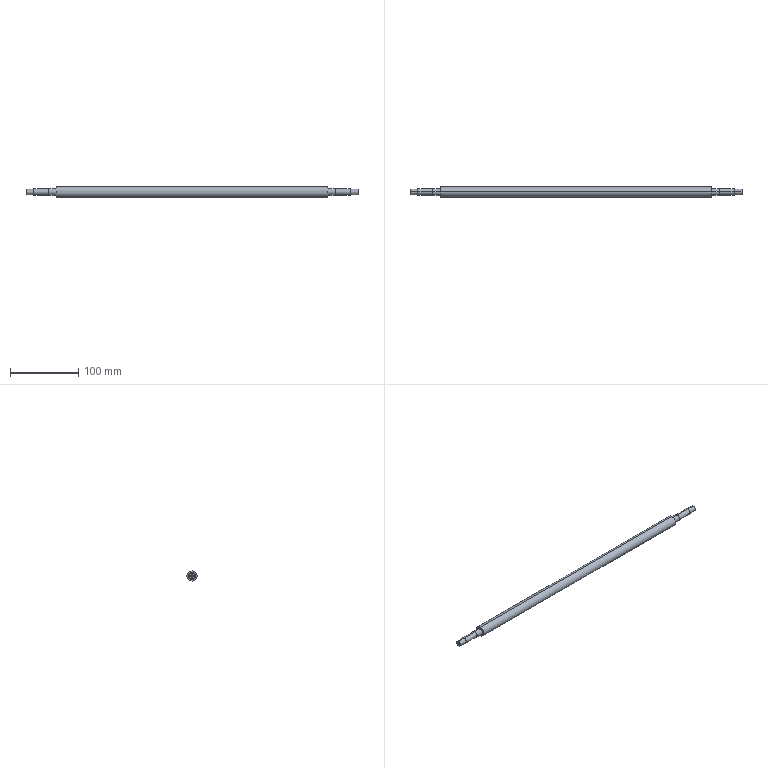Component | SolidWorks | PushRod3-1 | 1 solid | 28 faces | box 487 x 15 x 15 mm | volume 75810 mm3 | cylinder 18 | plane 10 | commonest cylinder face diameters 8 x4 3.3 x4 9 x4 10 x4 15 x2
STEP:
#1=COLOUR_RGB('',0.7922,0.8196,0.9333);
#2=FILL_AREA_STYLE_COLOUR('',#1);
#3=FILL_AREA_STYLE('',(#2));
#4=SURFACE_STYLE_FILL_AREA(#3);
#5=SURFACE_SIDE_STYLE('',(#4));
#6=SURFACE_STYLE_USAGE(.BOTH.,#5);
#7=PRESENTATION_STYLE_ASSIGNMENT((#6));
#8=CARTESIAN_POINT('',(9.587,5.032,2.961));
#9=VERTEX_POINT('',#8);
#10=CARTESIAN_POINT('',(9.587,5.032,3.276));
#11=VERTEX_POINT('',#10);
#12=CARTESIAN_POINT('',(9.587,5.032,3.119));
#13=DIRECTION('',(1.,0.,0.));
#14=DIRECTION('',(0.,0.,-1.));
#15=AXIS2_PLACEMENT_3D('',#12,#13,#14);
#16=CIRCLE('',#15,0.1575);
#17=EDGE_CURVE('',#9,#11,#16,.T.);
#18=ORIENTED_EDGE('',*,*,#17,.F.);
#19=CARTESIAN_POINT('',(9.134,5.032,2.961));
#20=VERTEX_POINT('',#19);
#21=CARTESIAN_POINT('',(9.587,5.032,2.961));
#22=DIRECTION('',(-1.,0.,0.));
#23=VECTOR('',#22,39.37);
#24=LINE('',#21,#23);
#25=EDGE_CURVE('',#9,#20,#24,.T.);
#26=ORIENTED_EDGE('',*,*,#25,.T.);
#27=CARTESIAN_POINT('',(9.134,5.032,3.276));
#28=VERTEX_POINT('',#27);
#29=CARTESIAN_POINT('',(9.134,5.032,3.119));
#30=DIRECTION('',(1.,0.,0.));
#31=DIRECTION('',(0.,0.,-1.));
#32=AXIS2_PLACEMENT_3D('',#29,#30,#31);
#33=CIRCLE('',#32,0.1575);
#34=EDGE_CURVE('',#20,#28,#33,.T.);
#35=ORIENTED_EDGE('',*,*,#34,.T.);
#36=CARTESIAN_POINT('',(9.587,5.032,3.276));
#37=DIRECTION('',(-1.,0.,0.));
#38=VECTOR('',#37,39.37);
#39=LINE('',#36,#38);
#40=EDGE_CURVE('',#11,#28,#39,.T.);
#41=ORIENTED_EDGE('',*,*,#40,.F.);
#42=EDGE_LOOP('',(#18,#26,#35,#41));
#43=FACE_OUTER_BOUND('',#42,.T.);
#44=CARTESIAN_POINT('',(9.587,5.032,3.119));
#45=DIRECTION('',(-1.,0.,0.));
#46=DIRECTION('',(0.,0.,1.));
#47=AXIS2_PLACEMENT_3D('',#44,#45,#46);
#48=CYLINDRICAL_SURFACE('',#47,0.1575);
#49=ADVANCED_FACE('',(#43),#48,.T.);
#50=CARTESIAN_POINT('',(9.114,5.032,3.184));
#51=VERTEX_POINT('',#50);
#52=CARTESIAN_POINT('',(9.114,5.032,3.054));
#53=VERTEX_POINT('',#52);
#54=CARTESIAN_POINT('',(9.114,5.032,3.119));
#55=DIRECTION('',(1.,0.,0.));
#56=DIRECTION('',(0.,0.,-1.));
#57=AXIS2_PLACEMENT_3D('',#54,#55,#56);
#58=CIRCLE('',#57,0.06496);
#59=EDGE_CURVE('',#51,#53,#58,.T.);
#60=ORIENTED_EDGE('',*,*,#59,.F.);
#61=CARTESIAN_POINT('',(9.587,5.032,3.184));
#62=VERTEX_POINT('',#61);
#63=CARTESIAN_POINT('',(9.114,5.032,3.184));
#64=DIRECTION('',(1.,0.,0.));
#65=VECTOR('',#64,39.37);
#66=LINE('',#63,#65);
#67=EDGE_CURVE('',#51,#62,#66,.T.);
#68=ORIENTED_EDGE('',*,*,#67,.T.);
#69=CARTESIAN_POINT('',(9.587,5.032,3.054));
#70=VERTEX_POINT('',#69);
#71=CARTESIAN_POINT('',(9.587,5.032,3.119));
#72=DIRECTION('',(1.,0.,0.));
#73=DIRECTION('',(0.,0.,-1.));
#74=AXIS2_PLACEMENT_3D('',#71,#72,#73);
#75=CIRCLE('',#74,0.06496);
#76=EDGE_CURVE('',#62,#70,#75,.T.);
#77=ORIENTED_EDGE('',*,*,#76,.T.);
#78=CARTESIAN_POINT('',(9.114,5.032,3.054));
#79=DIRECTION('',(1.,0.,0.));
#80=VECTOR('',#79,39.37);
#81=LINE('',#78,#80);
#82=EDGE_CURVE('',#53,#70,#81,.T.);
#83=ORIENTED_EDGE('',*,*,#82,.F.);
#84=EDGE_LOOP('',(#60,#68,#77,#83));
#85=FACE_OUTER_BOUND('',#84,.T.);
#86=CARTESIAN_POINT('',(9.114,5.032,3.119));
#87=DIRECTION('',(1.,0.,0.));
#88=DIRECTION('',(0.,0.,-1.));
#89=AXIS2_PLACEMENT_3D('',#86,#87,#88);
#90=CYLINDRICAL_SURFACE('',#89,0.06496);
#91=ADVANCED_FACE('',(#85),#90,.F.);
#92=CARTESIAN_POINT('',(8.268,5.032,3.296));
#93=VERTEX_POINT('',#92);
#94=CARTESIAN_POINT('',(8.268,5.032,2.941));
#95=VERTEX_POINT('',#94);
#96=CARTESIAN_POINT('',(8.268,5.032,3.119));
#97=DIRECTION('',(-1.,0.,0.));
#98=DIRECTION('',(0.,0.,1.));
#99=AXIS2_PLACEMENT_3D('',#96,#97,#98);
#100=CIRCLE('',#99,0.1772);
#101=EDGE_CURVE('',#93,#95,#100,.T.);
#102=ORIENTED_EDGE('',*,*,#101,.F.);
#103=CARTESIAN_POINT('',(9.134,5.032,3.296));
#104=VERTEX_POINT('',#103);
#105=CARTESIAN_POINT('',(8.228,5.032,3.296));
#106=DIRECTION('',(1.,0.,0.));
#107=VECTOR('',#106,39.37);
#108=LINE('',#105,#107);
#109=EDGE_CURVE('',#93,#104,#108,.T.);
#110=ORIENTED_EDGE('',*,*,#109,.T.);
#111=CARTESIAN_POINT('',(9.134,5.032,2.941));
#112=VERTEX_POINT('',#111);
#113=CARTESIAN_POINT('',(9.134,5.032,3.119));
#114=DIRECTION('',(1.,0.,0.));
#115=DIRECTION('',(0.,0.,-1.));
#116=AXIS2_PLACEMENT_3D('',#113,#114,#115);
#117=CIRCLE('',#116,0.1772);
#118=EDGE_CURVE('',#112,#104,#117,.T.);
#119=ORIENTED_EDGE('',*,*,#118,.F.);
#120=CARTESIAN_POINT('',(8.228,5.032,2.941));
#121=DIRECTION('',(1.,0.,0.));
#122=VECTOR('',#121,39.37);
#123=LINE('',#120,#122);
#124=EDGE_CURVE('',#95,#112,#123,.T.);
#125=ORIENTED_EDGE('',*,*,#124,.F.);
#126=EDGE_LOOP('',(#102,#110,#119,#125));
#127=FACE_OUTER_BOUND('',#126,.T.);
#128=CARTESIAN_POINT('',(8.228,5.032,3.119));
#129=DIRECTION('',(1.,0.,0.));
#130=DIRECTION('',(0.,0.,-1.));
#131=AXIS2_PLACEMENT_3D('',#128,#129,#130);
#132=CYLINDRICAL_SURFACE('',#131,0.1772);
#133=ADVANCED_FACE('',(#127),#132,.T.);
#134=CARTESIAN_POINT('',(8.268,5.032,3.315));
#135=VERTEX_POINT('',#134);
#136=CARTESIAN_POINT('',(8.268,5.032,2.922));
#137=VERTEX_POINT('',#136);
#138=CARTESIAN_POINT('',(8.268,5.032,3.119));
#139=DIRECTION('',(-1.,0.,0.));
#140=DIRECTION('',(0.,0.,1.));
#141=AXIS2_PLACEMENT_3D('',#138,#139,#140);
#142=CIRCLE('',#141,0.1969);
#143=EDGE_CURVE('',#135,#137,#142,.T.);
#144=ORIENTED_EDGE('',*,*,#143,.T.);
#145=CARTESIAN_POINT('',(7.835,5.032,2.922));
#146=VERTEX_POINT('',#145);
#147=CARTESIAN_POINT('',(9.134,5.032,2.922));
#148=DIRECTION('',(-1.,0.,0.));
#149=VECTOR('',#148,39.37);
#150=LINE('',#147,#149);
#151=EDGE_CURVE('',#137,#146,#150,.T.);
#152=ORIENTED_EDGE('',*,*,#151,.T.);
#153=CARTESIAN_POINT('',(7.835,5.032,3.315));
#154=VERTEX_POINT('',#153);
#155=CARTESIAN_POINT('',(7.835,5.032,3.119));
#156=DIRECTION('',(1.,0.,0.));
#157=DIRECTION('',(0.,0.,-1.));
#158=AXIS2_PLACEMENT_3D('',#155,#156,#157);
#159=CIRCLE('',#158,0.1969);
#160=EDGE_CURVE('',#146,#154,#159,.T.);
#161=ORIENTED_EDGE('',*,*,#160,.T.);
#162=CARTESIAN_POINT('',(9.134,5.032,3.315));
#163=DIRECTION('',(-1.,0.,0.));
#164=VECTOR('',#163,39.37);
#165=LINE('',#162,#164);
#166=EDGE_CURVE('',#135,#154,#165,.T.);
#167=ORIENTED_EDGE('',*,*,#166,.F.);
#168=EDGE_LOOP('',(#144,#152,#161,#167));
#169=FACE_OUTER_BOUND('',#168,.T.);
#170=CARTESIAN_POINT('',(9.134,5.032,3.119));
#171=DIRECTION('',(-1.,0.,0.));
#172=DIRECTION('',(0.,0.,1.));
#173=AXIS2_PLACEMENT_3D('',#170,#171,#172);
#174=CYLINDRICAL_SURFACE('',#173,0.1969);
#175=ADVANCED_FACE('',(#169),#174,.T.);
#176=CARTESIAN_POINT('',(7.835,5.032,2.823));
#177=VERTEX_POINT('',#176);
#178=CARTESIAN_POINT('',(7.835,5.032,3.414));
#179=VERTEX_POINT('',#178);
#180=CARTESIAN_POINT('',(7.835,5.032,3.119));
#181=DIRECTION('',(1.,0.,0.));
#182=DIRECTION('',(0.,0.,-1.));
#183=AXIS2_PLACEMENT_3D('',#180,#181,#182);
#184=CIRCLE('',#183,0.2953);
#185=EDGE_CURVE('',#177,#179,#184,.T.);
#186=ORIENTED_EDGE('',*,*,#185,.F.);
#187=CARTESIAN_POINT('',(-7.835,5.032,2.823));
#188=VERTEX_POINT('',#187);
#189=CARTESIAN_POINT('',(7.835,5.032,2.823));
#190=DIRECTION('',(-1.,0.,0.));
#191=VECTOR('',#190,39.37);
#192=LINE('',#189,#191);
#193=EDGE_CURVE('',#177,#188,#192,.T.);
#194=ORIENTED_EDGE('',*,*,#193,.T.);
#195=CARTESIAN_POINT('',(-7.835,5.032,3.414));
#196=VERTEX_POINT('',#195);
#197=CARTESIAN_POINT('',(-7.835,5.032,3.119));
#198=DIRECTION('',(1.,0.,0.));
#199=DIRECTION('',(0.,0.,-1.));
#200=AXIS2_PLACEMENT_3D('',#197,#198,#199);
#201=CIRCLE('',#200,0.2953);
#202=EDGE_CURVE('',#188,#196,#201,.T.);
#203=ORIENTED_EDGE('',*,*,#202,.T.);
#204=CARTESIAN_POINT('',(7.835,5.032,3.414));
#205=DIRECTION('',(-1.,0.,0.));
#206=VECTOR('',#205,39.37);
#207=LINE('',#204,#206);
#208=EDGE_CURVE('',#179,#196,#207,.T.);
#209=ORIENTED_EDGE('',*,*,#208,.F.);
#210=EDGE_LOOP('',(#186,#194,#203,#209));
#211=FACE_OUTER_BOUND('',#210,.T.);
#212=CARTESIAN_POINT('',(7.835,5.032,3.119));
#213=DIRECTION('',(-1.,0.,0.));
#214=DIRECTION('',(0.,0.,1.));
#215=AXIS2_PLACEMENT_3D('',#212,#213,#214);
#216=CYLINDRICAL_SURFACE('',#215,0.2953);
#217=ADVANCED_FACE('',(#211),#216,.T.);
#218=CARTESIAN_POINT('',(-8.268,5.032,2.922));
#219=VERTEX_POINT('',#218);
#220=CARTESIAN_POINT('',(-8.268,5.032,3.315));
#221=VERTEX_POINT('',#220);
#222=CARTESIAN_POINT('',(-8.268,5.032,3.119));
#223=DIRECTION('',(1.,0.,0.));
#224=DIRECTION('',(0.,0.,-1.));
#225=AXIS2_PLACEMENT_3D('',#222,#223,#224);
#226=CIRCLE('',#225,0.1969);
#227=EDGE_CURVE('',#219,#221,#226,.T.);
#228=ORIENTED_EDGE('',*,*,#227,.T.);
#229=CARTESIAN_POINT('',(-7.835,5.032,3.315));
#230=VERTEX_POINT('',#229);
#231=CARTESIAN_POINT('',(-9.134,5.032,3.315));
#232=DIRECTION('',(1.,0.,0.));
#233=VECTOR('',#232,39.37);
#234=LINE('',#231,#233);
#235=EDGE_CURVE('',#221,#230,#234,.T.);
#236=ORIENTED_EDGE('',*,*,#235,.T.);
#237=CARTESIAN_POINT('',(-7.835,5.032,2.922));
#238=VERTEX_POINT('',#237);
#239=CARTESIAN_POINT('',(-7.835,5.032,3.119));
#240=DIRECTION('',(-1.,0.,0.));
#241=DIRECTION('',(0.,0.,-1.));
#242=AXIS2_PLACEMENT_3D('',#239,#240,#241);
#243=CIRCLE('',#242,0.1969);
#244=EDGE_CURVE('',#230,#238,#243,.T.);
#245=ORIENTED_EDGE('',*,*,#244,.T.);
#246=CARTESIAN_POINT('',(-9.134,5.032,2.922));
#247=DIRECTION('',(1.,0.,0.));
#248=VECTOR('',#247,39.37);
#249=LINE('',#246,#248);
#250=EDGE_CURVE('',#219,#238,#249,.T.);
#251=ORIENTED_EDGE('',*,*,#250,.F.);
#252=EDGE_LOOP('',(#228,#236,#245,#251));
#253=FACE_OUTER_BOUND('',#252,.T.);
#254=CARTESIAN_POINT('',(-9.134,5.032,3.119));
#255=DIRECTION('',(1.,0.,0.));
#256=DIRECTION('',(0.,0.,-1.));
#257=AXIS2_PLACEMENT_3D('',#254,#255,#256);
#258=CYLINDRICAL_SURFACE('',#257,0.1969);
#259=ADVANCED_FACE('',(#253),#258,.T.);
#260=CARTESIAN_POINT('',(-9.134,5.032,3.296));
#261=VERTEX_POINT('',#260);
#262=CARTESIAN_POINT('',(-9.134,5.032,2.941));
#263=VERTEX_POINT('',#262);
#264=CARTESIAN_POINT('',(-9.134,5.032,3.119));
#265=DIRECTION('',(-1.,0.,0.));
#266=DIRECTION('',(0.,0.,1.));
#267=AXIS2_PLACEMENT_3D('',#264,#265,#266);
#268=CIRCLE('',#267,0.1772);
#269=EDGE_CURVE('',#261,#263,#268,.T.);
#270=ORIENTED_EDGE('',*,*,#269,.F.);
#271=CARTESIAN_POINT('',(-8.268,5.032,3.296));
#272=VERTEX_POINT('',#271);
#273=CARTESIAN_POINT('',(-9.213,5.032,3.296));
#274=DIRECTION('',(1.,0.,0.));
#275=VECTOR('',#274,39.37);
#276=LINE('',#273,#275);
#277=EDGE_CURVE('',#261,#272,#276,.T.);
#278=ORIENTED_EDGE('',*,*,#277,.T.);
#279=CARTESIAN_POINT('',(-8.268,5.032,2.941));
#280=VERTEX_POINT('',#279);
#281=CARTESIAN_POINT('',(-8.268,5.032,3.119));
#282=DIRECTION('',(1.,0.,0.));
#283=DIRECTION('',(0.,0.,-1.));
#284=AXIS2_PLACEMENT_3D('',#281,#282,#283);
#285=CIRCLE('',#284,0.1772);
#286=EDGE_CURVE('',#280,#272,#285,.T.);
#287=ORIENTED_EDGE('',*,*,#286,.F.);
#288=CARTESIAN_POINT('',(-9.213,5.032,2.941));
#289=DIRECTION('',(1.,0.,0.));
#290=VECTOR('',#289,39.37);
#291=LINE('',#288,#290);
#292=EDGE_CURVE('',#263,#280,#291,.T.);
#293=ORIENTED_EDGE('',*,*,#292,.F.);
#294=EDGE_LOOP('',(#270,#278,#287,#293));
#295=FACE_OUTER_BOUND('',#294,.T.);
#296=CARTESIAN_POINT('',(-9.213,5.032,3.119));
#297=DIRECTION('',(1.,0.,0.));
#298=DIRECTION('',(0.,0.,-1.));
#299=AXIS2_PLACEMENT_3D('',#296,#297,#298);
#300=CYLINDRICAL_SURFACE('',#299,0.1772);
#301=ADVANCED_FACE('',(#295),#300,.T.);
#302=CARTESIAN_POINT('',(-9.114,5.032,3.054));
#303=VERTEX_POINT('',#302);
#304=CARTESIAN_POINT('',(-9.114,5.032,3.184));
#305=VERTEX_POINT('',#304);
#306=CARTESIAN_POINT('',(-9.114,5.032,3.119));
#307=DIRECTION('',(-1.,0.,0.));
#308=DIRECTION('',(0.,0.,1.));
#309=AXIS2_PLACEMENT_3D('',#306,#307,#308);
#310=CIRCLE('',#309,0.06496);
#311=EDGE_CURVE('',#303,#305,#310,.T.);
#312=ORIENTED_EDGE('',*,*,#311,.F.);
#313=CARTESIAN_POINT('',(-9.587,5.032,3.054));
#314=VERTEX_POINT('',#313);
#315=CARTESIAN_POINT('',(-9.114,5.032,3.054));
#316=DIRECTION('',(-1.,0.,0.));
#317=VECTOR('',#316,39.37);
#318=LINE('',#315,#317);
#319=EDGE_CURVE('',#303,#314,#318,.T.);
#320=ORIENTED_EDGE('',*,*,#319,.T.);
#321=CARTESIAN_POINT('',(-9.587,5.032,3.184));
#322=VERTEX_POINT('',#321);
#323=CARTESIAN_POINT('',(-9.587,5.032,3.119));
#324=DIRECTION('',(-1.,0.,0.));
#325=DIRECTION('',(0.,0.,1.));
#326=AXIS2_PLACEMENT_3D('',#323,#324,#325);
#327=CIRCLE('',#326,0.06496);
#328=EDGE_CURVE('',#314,#322,#327,.T.);
#329=ORIENTED_EDGE('',*,*,#328,.T.);
#330=CARTESIAN_POINT('',(-9.114,5.032,3.184));
#331=DIRECTION('',(-1.,0.,0.));
#332=VECTOR('',#331,39.37);
#333=LINE('',#330,#332);
#334=EDGE_CURVE('',#305,#322,#333,.T.);
#335=ORIENTED_EDGE('',*,*,#334,.F.);
#336=EDGE_LOOP('',(#312,#320,#329,#335));
#337=FACE_OUTER_BOUND('',#336,.T.);
#338=CARTESIAN_POINT('',(-9.114,5.032,3.119));
#339=DIRECTION('',(-1.,0.,0.));
#340=DIRECTION('',(0.,0.,1.));
#341=AXIS2_PLACEMENT_3D('',#338,#339,#340);
#342=CYLINDRICAL_SURFACE('',#341,0.06496);
#343=ADVANCED_FACE('',(#337),#342,.F.);
#344=CARTESIAN_POINT('',(-9.587,5.032,3.276));
#345=VERTEX_POINT('',#344);
#346=CARTESIAN_POINT('',(-9.587,5.032,2.961));
#347=VERTEX_POINT('',#346);
#348=CARTESIAN_POINT('',(-9.587,5.032,3.119));
#349=DIRECTION('',(-1.,0.,0.));
#350=DIRECTION('',(0.,0.,1.));
#351=AXIS2_PLACEMENT_3D('',#348,#349,#350);
#352=CIRCLE('',#351,0.1575);
#353=EDGE_CURVE('',#345,#347,#352,.T.);
#354=ORIENTED_EDGE('',*,*,#353,.F.);
#355=CARTESIAN_POINT('',(-9.134,5.032,3.276));
#356=VERTEX_POINT('',#355);
#357=CARTESIAN_POINT('',(-9.587,5.032,3.276));
#358=DIRECTION('',(1.,0.,0.));
#359=VECTOR('',#358,39.37);
#360=LINE('',#357,#359);
#361=EDGE_CURVE('',#345,#356,#360,.T.);
#362=ORIENTED_EDGE('',*,*,#361,.T.);
#363=CARTESIAN_POINT('',(-9.134,5.032,2.961));
#364=VERTEX_POINT('',#363);
#365=CARTESIAN_POINT('',(-9.134,5.032,3.119));
#366=DIRECTION('',(-1.,0.,0.));
#367=DIRECTION('',(0.,0.,1.));
#368=AXIS2_PLACEMENT_3D('',#365,#366,#367);
#369=CIRCLE('',#368,0.1575);
#370=EDGE_CURVE('',#356,#364,#369,.T.);
#371=ORIENTED_EDGE('',*,*,#370,.T.);
#372=CARTESIAN_POINT('',(-9.587,5.032,2.961));
#373=DIRECTION('',(1.,0.,0.));
#374=VECTOR('',#373,39.37);
#375=LINE('',#372,#374);
#376=EDGE_CURVE('',#347,#364,#375,.T.);
#377=ORIENTED_EDGE('',*,*,#376,.F.);
#378=EDGE_LOOP('',(#354,#362,#371,#377));
#379=FACE_OUTER_BOUND('',#378,.T.);
#380=CARTESIAN_POINT('',(-9.587,5.032,3.119));
#381=DIRECTION('',(1.,0.,0.));
#382=DIRECTION('',(0.,0.,-1.));
#383=AXIS2_PLACEMENT_3D('',#380,#381,#382);
#384=CYLINDRICAL_SURFACE('',#383,0.1575);
#385=ADVANCED_FACE('',(#379),#384,.T.);
#386=CARTESIAN_POINT('',(-9.134,5.032,3.119));
#387=DIRECTION('',(-1.,0.,0.));
#388=DIRECTION('',(0.,0.,1.));
#389=AXIS2_PLACEMENT_3D('',#386,#387,#388);
#390=CIRCLE('',#389,0.1575);
#391=EDGE_CURVE('',#364,#356,#390,.T.);
#392=ORIENTED_EDGE('',*,*,#391,.F.);
#393=ORIENTED_EDGE('',*,*,#370,.F.);
#394=EDGE_LOOP('',(#392,#393));
#395=FACE_BOUND('',#394,.T.);
#396=CARTESIAN_POINT('',(-9.134,5.032,3.119));
#397=DIRECTION('',(-1.,0.,0.));
#398=DIRECTION('',(0.,0.,1.));
#399=AXIS2_PLACEMENT_3D('',#396,#397,#398);
#400=CIRCLE('',#399,0.1772);
#401=EDGE_CURVE('',#263,#261,#400,.T.);
#402=ORIENTED_EDGE('',*,*,#401,.T.);
#403=ORIENTED_EDGE('',*,*,#269,.T.);
#404=EDGE_LOOP('',(#402,#403));
#405=FACE_OUTER_BOUND('',#404,.T.);
#406=CARTESIAN_POINT('',(-9.134,5.032,3.119));
#407=DIRECTION('',(-1.,0.,0.));
#408=DIRECTION('',(0.,0.,1.));
#409=AXIS2_PLACEMENT_3D('',#406,#407,#408);
#410=PLANE('',#409);
#411=ADVANCED_FACE('',(#395,#405),#410,.T.);
#412=ORIENTED_EDGE('',*,*,#361,.F.);
#413=CARTESIAN_POINT('',(-9.587,5.032,3.119));
#414=DIRECTION('',(-1.,0.,0.));
#415=DIRECTION('',(0.,0.,1.));
#416=AXIS2_PLACEMENT_3D('',#413,#414,#415);
#417=CIRCLE('',#416,0.1575);
#418=EDGE_CURVE('',#347,#345,#417,.T.);
#419=ORIENTED_EDGE('',*,*,#418,.F.);
#420=ORIENTED_EDGE('',*,*,#376,.T.);
#421=ORIENTED_EDGE('',*,*,#391,.T.);
#422=EDGE_LOOP('',(#412,#419,#420,#421));
#423=FACE_OUTER_BOUND('',#422,.T.);
#424=CARTESIAN_POINT('',(-9.587,5.032,3.119));
#425=DIRECTION('',(1.,0.,0.));
#426=DIRECTION('',(0.,0.,-1.));
#427=AXIS2_PLACEMENT_3D('',#424,#425,#426);
#428=CYLINDRICAL_SURFACE('',#427,0.1575);
#429=ADVANCED_FACE('',(#423),#428,.T.);
#430=CARTESIAN_POINT('',(-9.587,5.032,3.119));
#431=DIRECTION('',(-1.,0.,0.));
#432=DIRECTION('',(0.,0.,1.));
#433=AXIS2_PLACEMENT_3D('',#430,#431,#432);
#434=CIRCLE('',#433,0.06496);
#435=EDGE_CURVE('',#322,#314,#434,.T.);
#436=ORIENTED_EDGE('',*,*,#435,.F.);
#437=ORIENTED_EDGE('',*,*,#328,.F.);
#438=EDGE_LOOP('',(#436,#437));
#439=FACE_BOUND('',#438,.T.);
#440=ORIENTED_EDGE('',*,*,#418,.T.);
#441=ORIENTED_EDGE('',*,*,#353,.T.);
#442=EDGE_LOOP('',(#440,#441));
#443=FACE_OUTER_BOUND('',#442,.T.);
#444=CARTESIAN_POINT('',(-9.587,5.032,3.119));
#445=DIRECTION('',(-1.,0.,0.));
#446=DIRECTION('',(0.,0.,1.));
#447=AXIS2_PLACEMENT_3D('',#444,#445,#446);
#448=PLANE('',#447);
#449=ADVANCED_FACE('',(#439,#443),#448,.T.);
#450=ORIENTED_EDGE('',*,*,#319,.F.);
#451=CARTESIAN_POINT('',(-9.114,5.032,3.119));
#452=DIRECTION('',(-1.,0.,0.));
#453=DIRECTION('',(0.,0.,1.));
#454=AXIS2_PLACEMENT_3D('',#451,#452,#453);
#455=CIRCLE('',#454,0.06496);
#456=EDGE_CURVE('',#305,#303,#455,.T.);
#457=ORIENTED_EDGE('',*,*,#456,.F.);
#458=ORIENTED_EDGE('',*,*,#334,.T.);
#459=ORIENTED_EDGE('',*,*,#435,.T.);
#460=EDGE_LOOP('',(#450,#457,#458,#459));
#461=FACE_OUTER_BOUND('',#460,.T.);
#462=CARTESIAN_POINT('',(-9.114,5.032,3.119));
#463=DIRECTION('',(-1.,0.,0.));
#464=DIRECTION('',(0.,0.,1.));
#465=AXIS2_PLACEMENT_3D('',#462,#463,#464);
#466=CYLINDRICAL_SURFACE('',#465,0.06496);
#467=ADVANCED_FACE('',(#461),#466,.F.);
#468=ORIENTED_EDGE('',*,*,#456,.T.);
#469=ORIENTED_EDGE('',*,*,#311,.T.);
#470=EDGE_LOOP('',(#468,#469));
#471=FACE_OUTER_BOUND('',#470,.T.);
#472=CARTESIAN_POINT('',(-9.114,5.032,3.119));
#473=DIRECTION('',(-1.,0.,0.));
#474=DIRECTION('',(0.,0.,1.));
#475=AXIS2_PLACEMENT_3D('',#472,#473,#474);
#476=PLANE('',#475);
#477=ADVANCED_FACE('',(#471),#476,.T.);
#478=ORIENTED_EDGE('',*,*,#286,.T.);
#479=CARTESIAN_POINT('',(-8.268,5.032,3.119));
#480=DIRECTION('',(1.,0.,0.));
#481=DIRECTION('',(0.,0.,-1.));
#482=AXIS2_PLACEMENT_3D('',#479,#480,#481);
#483=CIRCLE('',#482,0.1772);
#484=EDGE_CURVE('',#272,#280,#483,.T.);
#485=ORIENTED_EDGE('',*,*,#484,.T.);
#486=EDGE_LOOP('',(#478,#485));
#487=FACE_BOUND('',#486,.T.);
#488=ORIENTED_EDGE('',*,*,#227,.F.);
#489=CARTESIAN_POINT('',(-8.268,5.032,3.119));
#490=DIRECTION('',(1.,0.,0.));
#491=DIRECTION('',(0.,0.,-1.));
#492=AXIS2_PLACEMENT_3D('',#489,#490,#491);
#493=CIRCLE('',#492,0.1969);
#494=EDGE_CURVE('',#221,#219,#493,.T.);
#495=ORIENTED_EDGE('',*,*,#494,.F.);
#496=EDGE_LOOP('',(#488,#495));
#497=FACE_OUTER_BOUND('',#496,.T.);
#498=CARTESIAN_POINT('',(-8.268,5.032,3.119));
#499=DIRECTION('',(1.,0.,0.));
#500=DIRECTION('',(0.,0.,-1.));
#501=AXIS2_PLACEMENT_3D('',#498,#499,#500);
#502=PLANE('',#501);
#503=ADVANCED_FACE('',(#487,#497),#502,.F.);
#504=ORIENTED_EDGE('',*,*,#277,.F.);
#505=ORIENTED_EDGE('',*,*,#401,.F.);
#506=ORIENTED_EDGE('',*,*,#292,.T.);
#507=ORIENTED_EDGE('',*,*,#484,.F.);
#508=EDGE_LOOP('',(#504,#505,#506,#507));
#509=FACE_OUTER_BOUND('',#508,.T.);
#510=CARTESIAN_POINT('',(-9.213,5.032,3.119));
#511=DIRECTION('',(1.,0.,0.));
#512=DIRECTION('',(0.,0.,-1.));
#513=AXIS2_PLACEMENT_3D('',#510,#511,#512);
#514=CYLINDRICAL_SURFACE('',#513,0.1772);
#515=ADVANCED_FACE('',(#509),#514,.T.);
#516=CARTESIAN_POINT('',(-7.835,5.032,3.119));
#517=DIRECTION('',(1.,0.,0.));
#518=DIRECTION('',(0.,0.,-1.));
#519=AXIS2_PLACEMENT_3D('',#516,#517,#518);
#520=CIRCLE('',#519,0.2953);
#521=EDGE_CURVE('',#196,#188,#520,.T.);
#522=ORIENTED_EDGE('',*,*,#521,.F.);
#523=ORIENTED_EDGE('',*,*,#202,.F.);
#524=EDGE_LOOP('',(#522,#523));
#525=FACE_OUTER_BOUND('',#524,.T.);
#526=CARTESIAN_POINT('',(-7.835,5.032,3.119));
#527=DIRECTION('',(-1.,0.,0.));
#528=DIRECTION('',(0.,0.,-1.));
#529=AXIS2_PLACEMENT_3D('',#526,#527,#528);
#530=CIRCLE('',#529,0.1969);
#531=EDGE_CURVE('',#238,#230,#530,.T.);
#532=ORIENTED_EDGE('',*,*,#531,.F.);
#533=ORIENTED_EDGE('',*,*,#244,.F.);
#534=EDGE_LOOP('',(#532,#533));
#535=FACE_BOUND('',#534,.T.);
#536=CARTESIAN_POINT('',(-7.835,5.032,3.119));
#537=DIRECTION('',(1.,0.,0.));
#538=DIRECTION('',(0.,0.,-1.));
#539=AXIS2_PLACEMENT_3D('',#536,#537,#538);
#540=PLANE('',#539);
#541=ADVANCED_FACE('',(#525,#535),#540,.F.);
#542=ORIENTED_EDGE('',*,*,#235,.F.);
#543=ORIENTED_EDGE('',*,*,#494,.T.);
#544=ORIENTED_EDGE('',*,*,#250,.T.);
#545=ORIENTED_EDGE('',*,*,#531,.T.);
#546=EDGE_LOOP('',(#542,#543,#544,#545));
#547=FACE_OUTER_BOUND('',#546,.T.);
#548=CARTESIAN_POINT('',(-9.134,5.032,3.119));
#549=DIRECTION('',(1.,0.,0.));
#550=DIRECTION('',(0.,0.,-1.));
#551=AXIS2_PLACEMENT_3D('',#548,#549,#550);
#552=CYLINDRICAL_SURFACE('',#551,0.1969);
#553=ADVANCED_FACE('',(#547),#552,.T.);
#554=ORIENTED_EDGE('',*,*,#193,.F.);
#555=CARTESIAN_POINT('',(7.835,5.032,3.119));
#556=DIRECTION('',(1.,0.,0.));
#557=DIRECTION('',(0.,0.,-1.));
#558=AXIS2_PLACEMENT_3D('',#555,#556,#557);
#559=CIRCLE('',#558,0.2953);
#560=EDGE_CURVE('',#179,#177,#559,.T.);
#561=ORIENTED_EDGE('',*,*,#560,.F.);
#562=ORIENTED_EDGE('',*,*,#208,.T.);
#563=ORIENTED_EDGE('',*,*,#521,.T.);
#564=EDGE_LOOP('',(#554,#561,#562,#563));
#565=FACE_OUTER_BOUND('',#564,.T.);
#566=CARTESIAN_POINT('',(7.835,5.032,3.119));
#567=DIRECTION('',(-1.,0.,0.));
#568=DIRECTION('',(0.,0.,1.));
#569=AXIS2_PLACEMENT_3D('',#566,#567,#568);
#570=CYLINDRICAL_SURFACE('',#569,0.2953);
#571=ADVANCED_FACE('',(#565),#570,.T.);
#572=ORIENTED_EDGE('',*,*,#560,.T.);
#573=ORIENTED_EDGE('',*,*,#185,.T.);
#574=EDGE_LOOP('',(#572,#573));
#575=FACE_OUTER_BOUND('',#574,.T.);
#576=CARTESIAN_POINT('',(7.835,5.032,3.119));
#577=DIRECTION('',(1.,0.,0.));
#578=DIRECTION('',(0.,0.,-1.));
#579=AXIS2_PLACEMENT_3D('',#576,#577,#578);
#580=CIRCLE('',#579,0.1969);
#581=EDGE_CURVE('',#154,#146,#580,.T.);
#582=ORIENTED_EDGE('',*,*,#581,.F.);
#583=ORIENTED_EDGE('',*,*,#160,.F.);
#584=EDGE_LOOP('',(#582,#583));
#585=FACE_BOUND('',#584,.T.);
#586=CARTESIAN_POINT('',(7.835,5.032,3.119));
#587=DIRECTION('',(1.,0.,0.));
#588=DIRECTION('',(0.,0.,-1.));
#589=AXIS2_PLACEMENT_3D('',#586,#587,#588);
#590=PLANE('',#589);
#591=ADVANCED_FACE('',(#575,#585),#590,.T.);
#592=ORIENTED_EDGE('',*,*,#151,.F.);
#593=CARTESIAN_POINT('',(8.268,5.032,3.119));
#594=DIRECTION('',(-1.,0.,0.));
#595=DIRECTION('',(0.,0.,1.));
#596=AXIS2_PLACEMENT_3D('',#593,#594,#595);
#597=CIRCLE('',#596,0.1969);
#598=EDGE_CURVE('',#137,#135,#597,.T.);
#599=ORIENTED_EDGE('',*,*,#598,.T.);
#600=ORIENTED_EDGE('',*,*,#166,.T.);
#601=ORIENTED_EDGE('',*,*,#581,.T.);
#602=EDGE_LOOP('',(#592,#599,#600,#601));
#603=FACE_OUTER_BOUND('',#602,.T.);
#604=CARTESIAN_POINT('',(9.134,5.032,3.119));
#605=DIRECTION('',(-1.,0.,0.));
#606=DIRECTION('',(0.,0.,1.));
#607=AXIS2_PLACEMENT_3D('',#604,#605,#606);
#608=CYLINDRICAL_SURFACE('',#607,0.1969);
#609=ADVANCED_FACE('',(#603),#608,.T.);
#610=CARTESIAN_POINT('',(8.268,5.032,3.119));
#611=DIRECTION('',(-1.,0.,0.));
#612=DIRECTION('',(0.,0.,1.));
#613=AXIS2_PLACEMENT_3D('',#610,#611,#612);
#614=CIRCLE('',#613,0.1772);
#615=EDGE_CURVE('',#95,#93,#614,.T.);
#616=ORIENTED_EDGE('',*,*,#615,.T.);
#617=ORIENTED_EDGE('',*,*,#101,.T.);
#618=EDGE_LOOP('',(#616,#617));
#619=FACE_BOUND('',#618,.T.);
#620=ORIENTED_EDGE('',*,*,#143,.F.);
#621=ORIENTED_EDGE('',*,*,#598,.F.);
#622=EDGE_LOOP('',(#620,#621));
#623=FACE_OUTER_BOUND('',#622,.T.);
#624=CARTESIAN_POINT('',(8.268,5.032,3.119));
#625=DIRECTION('',(-1.,0.,0.));
#626=DIRECTION('',(0.,0.,1.));
#627=AXIS2_PLACEMENT_3D('',#624,#625,#626);
#628=PLANE('',#627);
#629=ADVANCED_FACE('',(#619,#623),#628,.F.);
#630=ORIENTED_EDGE('',*,*,#109,.F.);
#631=ORIENTED_EDGE('',*,*,#615,.F.);
#632=ORIENTED_EDGE('',*,*,#124,.T.);
#633=CARTESIAN_POINT('',(9.134,5.032,3.119));
#634=DIRECTION('',(1.,0.,0.));
#635=DIRECTION('',(0.,0.,-1.));
#636=AXIS2_PLACEMENT_3D('',#633,#634,#635);
#637=CIRCLE('',#636,0.1772);
#638=EDGE_CURVE('',#104,#112,#637,.T.);
#639=ORIENTED_EDGE('',*,*,#638,.F.);
#640=EDGE_LOOP('',(#630,#631,#632,#639));
#641=FACE_OUTER_BOUND('',#640,.T.);
#642=CARTESIAN_POINT('',(8.228,5.032,3.119));
#643=DIRECTION('',(1.,0.,0.));
#644=DIRECTION('',(0.,0.,-1.));
#645=AXIS2_PLACEMENT_3D('',#642,#643,#644);
#646=CYLINDRICAL_SURFACE('',#645,0.1772);
#647=ADVANCED_FACE('',(#641),#646,.T.);
#648=CARTESIAN_POINT('',(9.114,5.032,3.119));
#649=DIRECTION('',(1.,0.,0.));
#650=DIRECTION('',(0.,0.,-1.));
#651=AXIS2_PLACEMENT_3D('',#648,#649,#650);
#652=CIRCLE('',#651,0.06496);
#653=EDGE_CURVE('',#53,#51,#652,.T.);
#654=ORIENTED_EDGE('',*,*,#653,.T.);
#655=ORIENTED_EDGE('',*,*,#59,.T.);
#656=EDGE_LOOP('',(#654,#655));
#657=FACE_OUTER_BOUND('',#656,.T.);
#658=CARTESIAN_POINT('',(9.114,5.032,3.119));
#659=DIRECTION('',(1.,0.,0.));
#660=DIRECTION('',(0.,0.,-1.));
#661=AXIS2_PLACEMENT_3D('',#658,#659,#660);
#662=PLANE('',#661);
#663=ADVANCED_FACE('',(#657),#662,.T.);
#664=ORIENTED_EDGE('',*,*,#67,.F.);
#665=ORIENTED_EDGE('',*,*,#653,.F.);
#666=ORIENTED_EDGE('',*,*,#82,.T.);
#667=CARTESIAN_POINT('',(9.587,5.032,3.119));
#668=DIRECTION('',(1.,0.,0.));
#669=DIRECTION('',(0.,0.,-1.));
#670=AXIS2_PLACEMENT_3D('',#667,#668,#669);
#671=CIRCLE('',#670,0.06496);
#672=EDGE_CURVE('',#70,#62,#671,.T.);
#673=ORIENTED_EDGE('',*,*,#672,.T.);
#674=EDGE_LOOP('',(#664,#665,#666,#673));
#675=FACE_OUTER_BOUND('',#674,.T.);
#676=CARTESIAN_POINT('',(9.114,5.032,3.119));
#677=DIRECTION('',(1.,0.,0.));
#678=DIRECTION('',(0.,0.,-1.));
#679=AXIS2_PLACEMENT_3D('',#676,#677,#678);
#680=CYLINDRICAL_SURFACE('',#679,0.06496);
#681=ADVANCED_FACE('',(#675),#680,.F.);
#682=ORIENTED_EDGE('',*,*,#672,.F.);
#683=ORIENTED_EDGE('',*,*,#76,.F.);
#684=EDGE_LOOP('',(#682,#683));
#685=FACE_BOUND('',#684,.T.);
#686=CARTESIAN_POINT('',(9.587,5.032,3.119));
#687=DIRECTION('',(1.,0.,0.));
#688=DIRECTION('',(0.,0.,-1.));
#689=AXIS2_PLACEMENT_3D('',#686,#687,#688);
#690=CIRCLE('',#689,0.1575);
#691=EDGE_CURVE('',#11,#9,#690,.T.);
#692=ORIENTED_EDGE('',*,*,#691,.T.);
#693=ORIENTED_EDGE('',*,*,#17,.T.);
#694=EDGE_LOOP('',(#692,#693));
#695=FACE_OUTER_BOUND('',#694,.T.);
#696=CARTESIAN_POINT('',(9.587,5.032,3.119));
#697=DIRECTION('',(1.,0.,0.));
#698=DIRECTION('',(0.,0.,-1.));
#699=AXIS2_PLACEMENT_3D('',#696,#697,#698);
#700=PLANE('',#699);
#701=ADVANCED_FACE('',(#685,#695),#700,.T.);
#702=ORIENTED_EDGE('',*,*,#25,.F.);
#703=ORIENTED_EDGE('',*,*,#691,.F.);
#704=ORIENTED_EDGE('',*,*,#40,.T.);
#705=CARTESIAN_POINT('',(9.134,5.032,3.119));
#706=DIRECTION('',(1.,0.,0.));
#707=DIRECTION('',(0.,0.,-1.));
#708=AXIS2_PLACEMENT_3D('',#705,#706,#707);
#709=CIRCLE('',#708,0.1575);
#710=EDGE_CURVE('',#28,#20,#709,.T.);
#711=ORIENTED_EDGE('',*,*,#710,.T.);
#712=EDGE_LOOP('',(#702,#703,#704,#711));
#713=FACE_OUTER_BOUND('',#712,.T.);
#714=CARTESIAN_POINT('',(9.587,5.032,3.119));
#715=DIRECTION('',(-1.,0.,0.));
#716=DIRECTION('',(0.,0.,1.));
#717=AXIS2_PLACEMENT_3D('',#714,#715,#716);
#718=CYLINDRICAL_SURFACE('',#717,0.1575);
#719=ADVANCED_FACE('',(#713),#718,.T.);
#720=ORIENTED_EDGE('',*,*,#710,.F.);
#721=ORIENTED_EDGE('',*,*,#34,.F.);
#722=EDGE_LOOP('',(#720,#721));
#723=FACE_BOUND('',#722,.T.);
#724=ORIENTED_EDGE('',*,*,#118,.T.);
#725=ORIENTED_EDGE('',*,*,#638,.T.);
#726=EDGE_LOOP('',(#724,#725));
#727=FACE_OUTER_BOUND('',#726,.T.);
#728=CARTESIAN_POINT('',(9.134,5.032,3.119));
#729=DIRECTION('',(1.,0.,0.));
#730=DIRECTION('',(0.,0.,-1.));
#731=AXIS2_PLACEMENT_3D('',#728,#729,#730);
#732=PLANE('',#731);
#733=ADVANCED_FACE('',(#723,#727),#732,.T.);
#734=CLOSED_SHELL('',(#49,#91,#133,#175,#217,#259,#301,#343,#385,#411,#429,#449,#467,#477,#503,#515,#541,#553,#571,#591,#609,#629,#647,#663,#681,#701,#719,#733));
#735=MANIFOLD_SOLID_BREP('',#734);
#736=STYLED_ITEM('',(#7),#735);
#737=(LENGTH_UNIT()NAMED_UNIT(*)SI_UNIT($,.METRE.));
#738=LENGTH_MEASURE_WITH_UNIT(LENGTH_MEASURE(0.0254),#737);
#739=DIMENSIONAL_EXPONENTS(1.,0.,0.,0.,0.,0.,0.);
#740=(CONVERSION_BASED_UNIT('',#738)LENGTH_UNIT()NAMED_UNIT(#739));
#741=UNCERTAINTY_MEASURE_WITH_UNIT(LENGTH_MEASURE(0.00001),#740,'','');
#742=(NAMED_UNIT(*)PLANE_ANGLE_UNIT()SI_UNIT($,.RADIAN.));
#743=(NAMED_UNIT(*)SI_UNIT($,.STERADIAN.)SOLID_ANGLE_UNIT());
#744=(GEOMETRIC_REPRESENTATION_CONTEXT(3)GLOBAL_UNCERTAINTY_ASSIGNED_CONTEXT((#741))GLOBAL_UNIT_ASSIGNED_CONTEXT((#740,#742,#743))REPRESENTATION_CONTEXT('',''));
#745=MECHANICAL_DESIGN_GEOMETRIC_PRESENTATION_REPRESENTATION('',(#736),#744);
#746=CARTESIAN_POINT('',(0.,0.,0.));
#747=DIRECTION('',(0.,0.,1.));
#748=DIRECTION('',(1.,0.,0.));
#749=AXIS2_PLACEMENT_3D('',#746,#747,#748);
#750=(LENGTH_UNIT()NAMED_UNIT(*)SI_UNIT($,.METRE.));
#751=LENGTH_MEASURE_WITH_UNIT(LENGTH_MEASURE(0.0254),#750);
#752=DIMENSIONAL_EXPONENTS(1.,0.,0.,0.,0.,0.,0.);
#753=(CONVERSION_BASED_UNIT('',#751)LENGTH_UNIT()NAMED_UNIT(#752));
#754=UNCERTAINTY_MEASURE_WITH_UNIT(LENGTH_MEASURE(0.00001),#753,'','');
#755=(NAMED_UNIT(*)PLANE_ANGLE_UNIT()SI_UNIT($,.RADIAN.));
#756=(NAMED_UNIT(*)SI_UNIT($,.STERADIAN.)SOLID_ANGLE_UNIT());
#757=(GEOMETRIC_REPRESENTATION_CONTEXT(3)GLOBAL_UNCERTAINTY_ASSIGNED_CONTEXT((#754))GLOBAL_UNIT_ASSIGNED_CONTEXT((#753,#755,#756))REPRESENTATION_CONTEXT('',''));
#758=ADVANCED_BREP_SHAPE_REPRESENTATION('',(#735,#749),#757);
#759=PRESENTATION_LAYER_ASSIGNMENT('','',(#736));